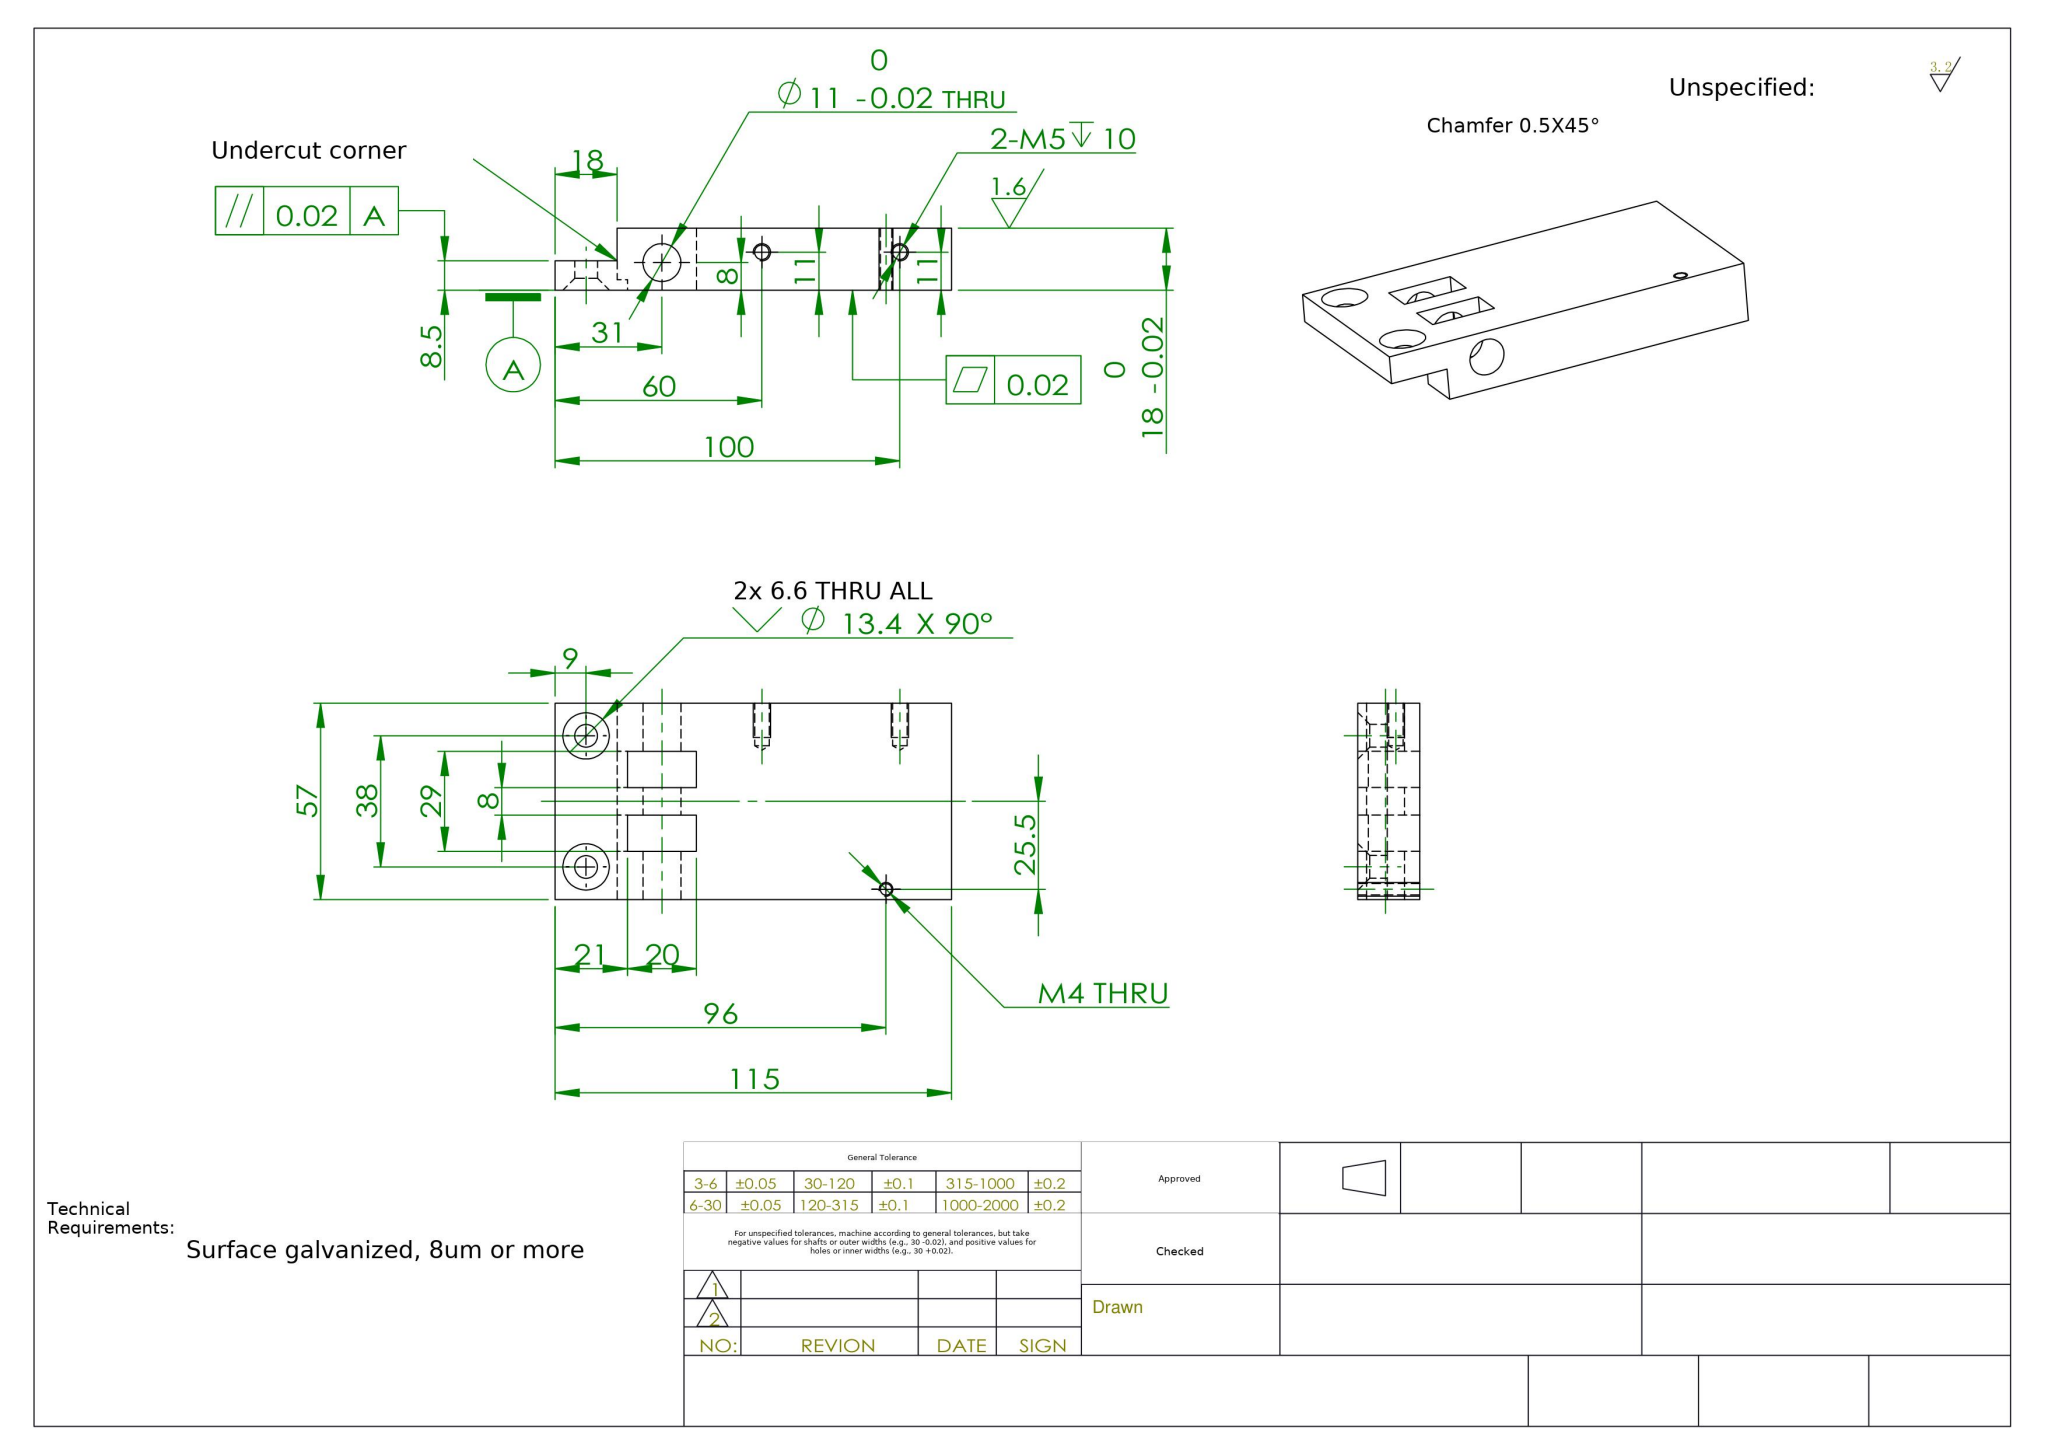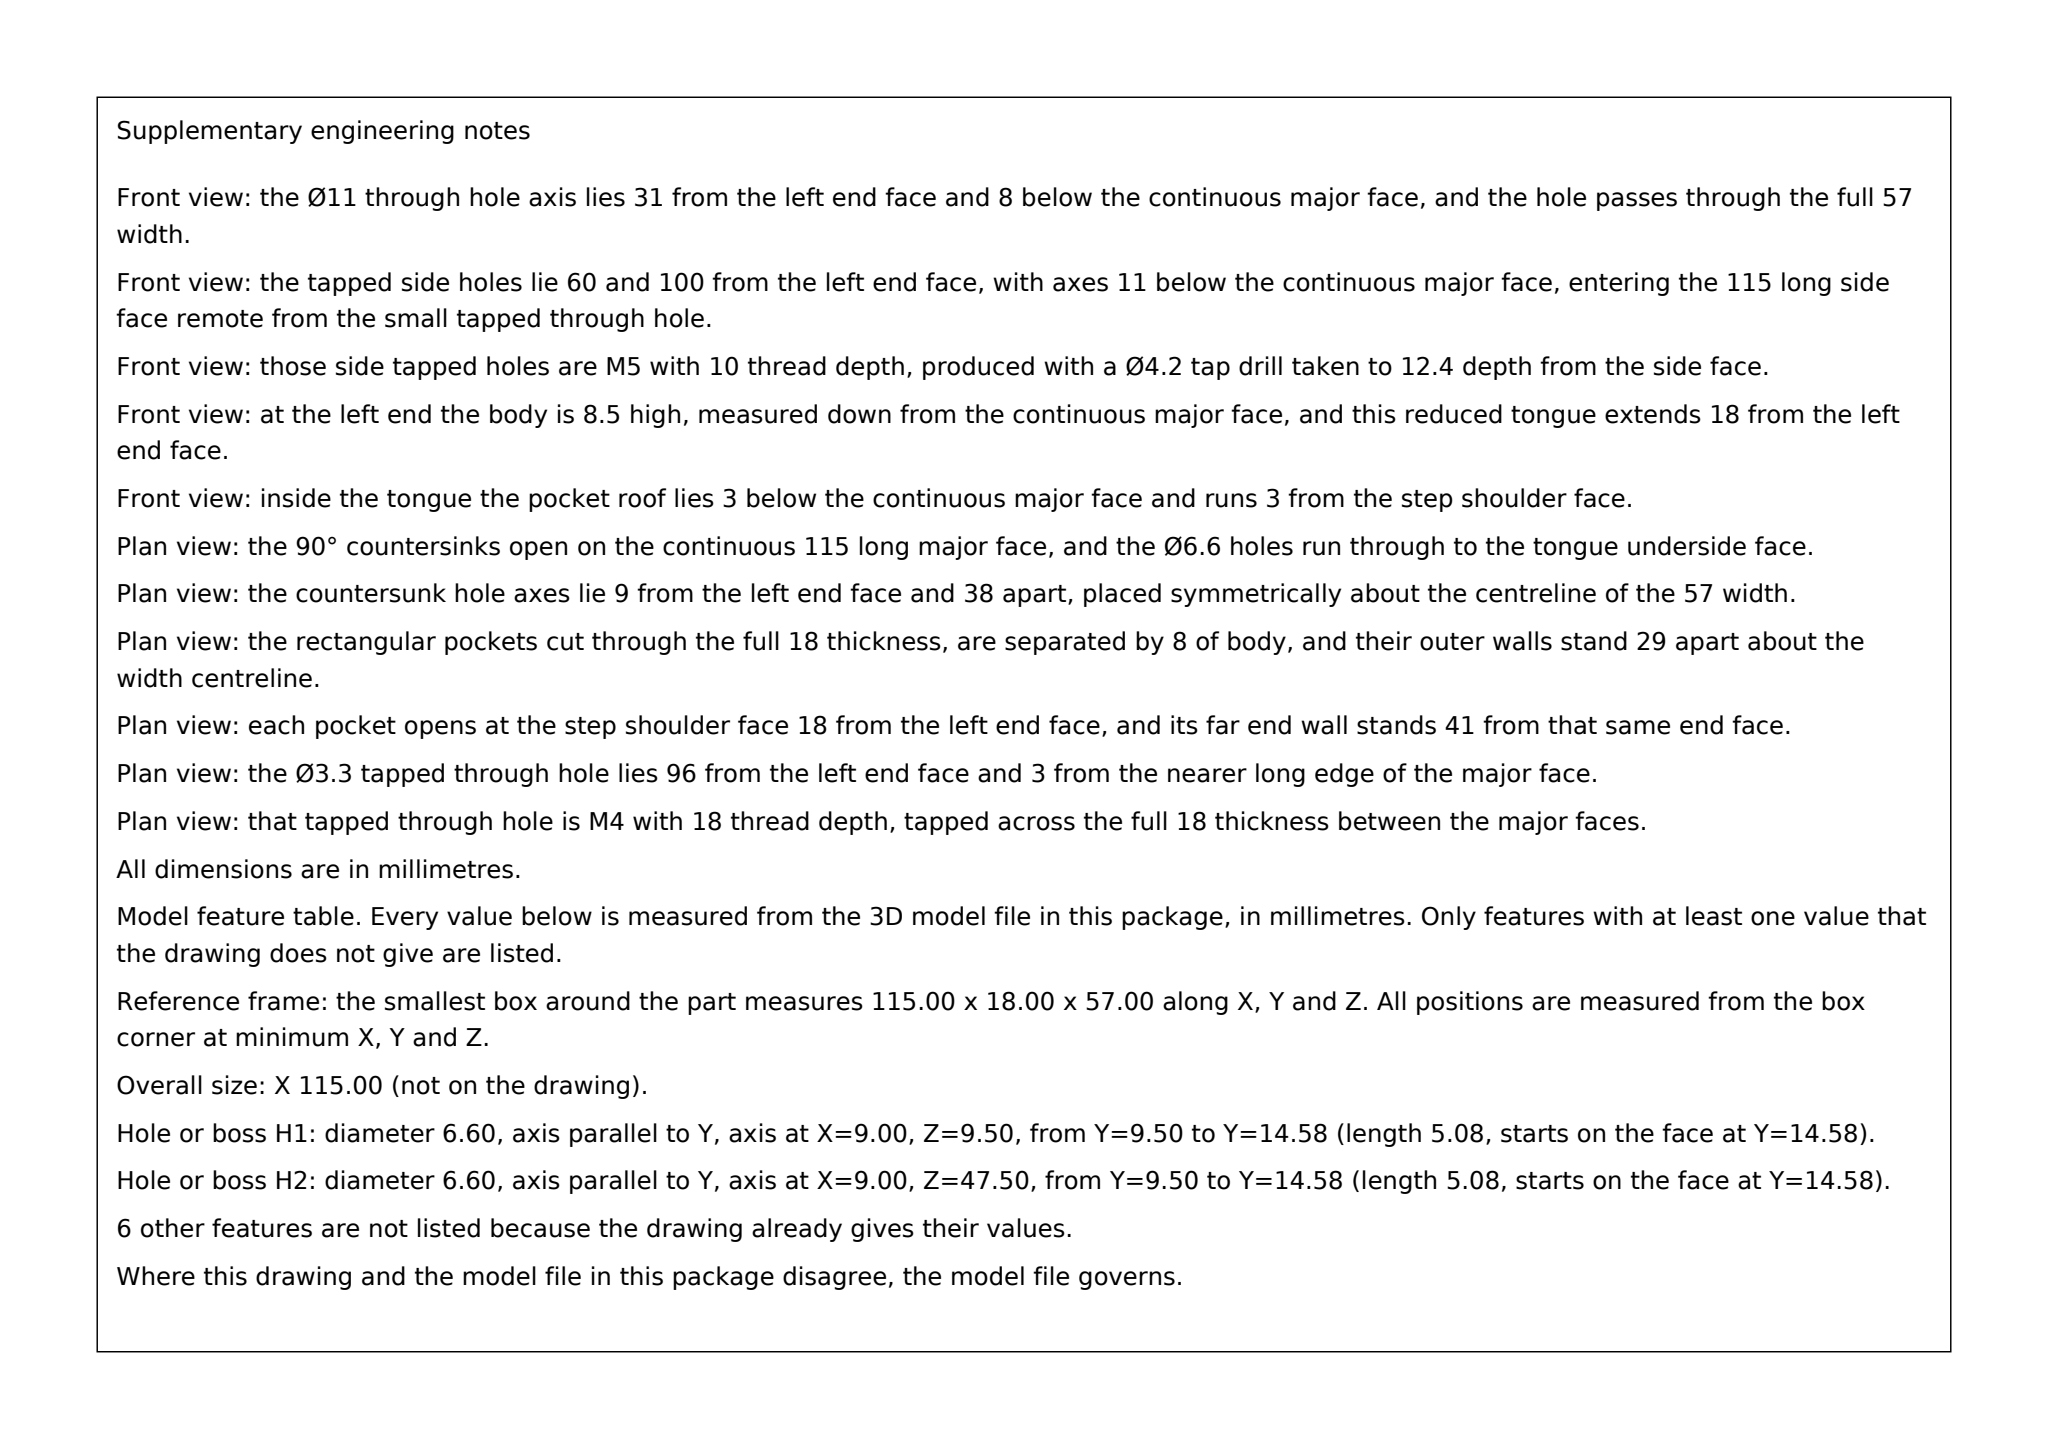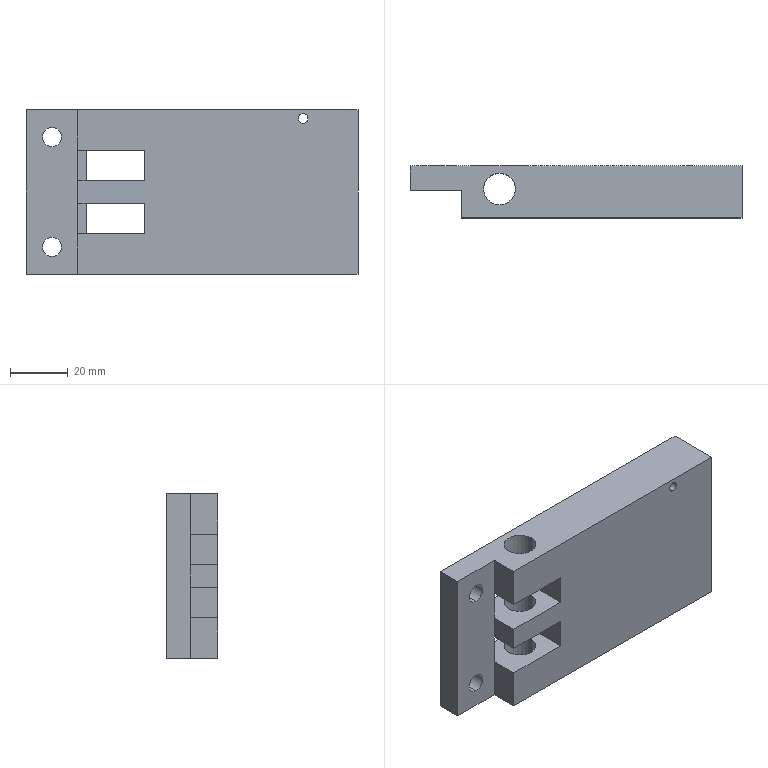Part | SolidWorks | mm | 1 solid | 46 faces | box 115 x 18 x 57 mm | volume 94900 mm3 | plane 22 | cylinder 16 | cone 8 | commonest cylinder face diameters 11 x6 4.2 x4 6.6 x4 3.3 x2
Drawing notes:
2X POCKET 20 LG X 10.5 WIDE, 8 APART, SYM ABT CL, 3 DP | from the solid: z-planes 14/24.5 and 32.5/43 (10.5 wide each, 8 between inner edges, 29 over outer edges); x-planes 21 & 41 (20 lg); y-plane 15 vs top y=18 (3 dp)
2X SLOT 10.5 WIDE X 23 LONG (FROM X=18 TO X=41 OFF LEFT END FACE), THRU FULL 18 THICKNESS (NOT A 3 DEEP POCKET); SLOT SIDE WALLS AT 14.0 AND 24.5, AND AT 32.5 AND 43.0 FROM BOTTOM EDGE (10.5 WIDE EACH, 8 APART, SYM ABOUT 57 WIDTH CL) | from the solid: axis_planes z=14.0 / z=24.5 / z=32.5 / z=43.0, extent x[18,41] y[0,18]; axis_plane x=41 extent y[0,18] z[14,24.5] and z[32.5,43]
2X UNDERCUT CORNER RELIEF AT SLOT MOUTH: 3 LONG (X=18 TO 21) X 3 HIGH (Y=15 TO TOP FACE Y=18), FULL 10.5 SLOT WIDTH; EXPOSED STEP FACE AT X=18 RUNS Y=9.5 TO 15 | from the solid: axis_planes x=21 extent y[15,18] z[14,24.5]/z[32.5,43] (area 31); y=15 extent x[18,21] same z ranges; x=18 extent y[9.5,15] (area 58)
SLOTS INTERRUPT THE Ø11 BORE: BORE IS CONTINUOUS ONLY Z=0-14, 24.5-32.5 AND 43-57, AXIS AT X=31, Y=10 FROM BOTTOM FACE | from the solid: cylinders dia 11.0 axis z at [31.0,10.0] from 0-14, 24.5-32.5, 43-57
build123d program:
from build123d import *

# Parameters (mm, degrees)
SKETCH1_W                                            = 115
SKETCH1_H                                            = 57
EXTRUDE1_DEPTH                                       = 9
SKETCH2_W                                            = 18
SKETCH2_H                                            = 9.5
CUT_EXTRUDE1_DEPTH                                   = 82.463
SKETCH3_W                                            = 20
SKETCH3_H                                            = 10.5
CUT_EXTRUDE2_DEPTH                                   = 67.652
SKETCH4_W                                            = 3
SKETCH4_H                                            = 10.5
CUT_EXTRUDE3_DEPTH                                   = 15
M6_HEXAGON_COUNTERSUNK_SCREW_COUNTERSUNK_D           = 6.6
M6_HEXAGON_COUNTERSUNK_SCREW_COUNTERSUNK_CSINK_D     = 13.44
M6_HEXAGON_COUNTERSUNK_SCREW_COUNTERSUNK_CSINK_ANGLE = 90
SKETCH8_R                                            = 5.5
CUT_EXTRUDE4_DEPTH                                   = 82.463
M5_TAPPED_HOLE1_D                                    = 4.2
M5_TAPPED_HOLE1_DEPTH                                = 12.4
M5_TAPPED_HOLE1_TIP                                  = 1.262
M4_TAPPED_HOLE1_D                                    = 3.3


with BuildPart() as part:
    # Sketch1 → Extrude1 (new, symmetric)
    with BuildSketch(Plane(origin=(0, 0, 0), x_dir=(1, 0, 0), z_dir=(0, 1, 0))):
        Rectangle(SKETCH1_W, SKETCH1_H)
    extrude(amount=EXTRUDE1_DEPTH, both=True)

    # Sketch2 → Cut-Extrude1 (cut, through all)
    with BuildSketch(Plane.XY.offset(28.5)):
        with Locations((-48.5, -4.25)):
            Rectangle(SKETCH2_W, SKETCH2_H)
    extrude(amount=-CUT_EXTRUDE1_DEPTH, mode=Mode.SUBTRACT)

    # Sketch3 → Cut-Extrude2 (cut, through all)
    with BuildSketch(Plane(origin=(0, 9, 0), x_dir=(1, 0, 0), z_dir=(0, 1, 0))):
        with Locations((-26.5, 9.25)):
            Rectangle(SKETCH3_W, SKETCH3_H)
        with Locations((-26.5, -9.25)):
            Rectangle(SKETCH3_W, SKETCH3_H)
    extrude(amount=-CUT_EXTRUDE2_DEPTH, mode=Mode.SUBTRACT)

    # Sketch4 → Cut-Extrude3 (cut)
    with BuildSketch(Plane.XZ.offset(9)):
        with Locations((-38, 9.25)):
            Rectangle(SKETCH4_W, SKETCH4_H)
        with Locations((-38, -9.25)):
            Rectangle(SKETCH4_W, SKETCH4_H)
    extrude(amount=-CUT_EXTRUDE3_DEPTH, mode=Mode.SUBTRACT)

    # M6 Hexagon Countersunk Screw Countersunk (through all)
    with Locations(Plane(origin=(0, 9, 0), x_dir=(-1, 0, 0), z_dir=(0, 1, 0))):
        with Locations((48.5, -19), (48.5, 19)):
            CounterSinkHole(M6_HEXAGON_COUNTERSUNK_SCREW_COUNTERSUNK_D / 2, M6_HEXAGON_COUNTERSUNK_SCREW_COUNTERSUNK_CSINK_D / 2, counter_sink_angle=M6_HEXAGON_COUNTERSUNK_SCREW_COUNTERSUNK_CSINK_ANGLE)

    # Sketch8 → Cut-Extrude4 (cut, through all)
    with BuildSketch(Plane.XY.offset(28.5)):
        with Locations((-26.5, 1)):
            Circle(SKETCH8_R)
    extrude(amount=-CUT_EXTRUDE4_DEPTH, mode=Mode.SUBTRACT)

    # M5 Tapped Hole1
    with Locations(Plane(origin=(0, 0, -28.5), x_dir=(-1, 0, 0), z_dir=(0, 0, -1))):
        with Locations((-42.5, -2), (-2.5, -2)):
            Hole(M5_TAPPED_HOLE1_D / 2, depth=M5_TAPPED_HOLE1_DEPTH)
            with Locations((0, 0, -(M5_TAPPED_HOLE1_DEPTH + M5_TAPPED_HOLE1_TIP / 2))):  # 118° drill point
                Cone(0, M5_TAPPED_HOLE1_D / 2, M5_TAPPED_HOLE1_TIP, mode=Mode.SUBTRACT)

    # M4 Tapped Hole1 (through all)
    with Locations(Plane(origin=(0, 9, 0), x_dir=(-1, 0, 0), z_dir=(0, 1, 0))):
        with Locations((-38.5, 25.5)):
            Hole(M4_TAPPED_HOLE1_D / 2)


solid = part.part